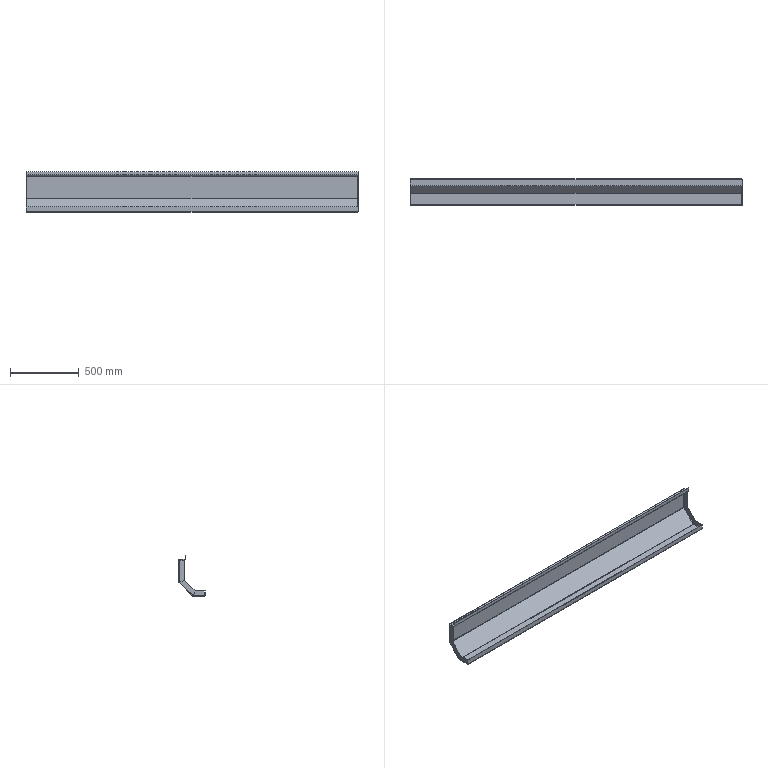Component | NX | UPPER_RIGHT_CROSSBEAM | 1 solid | 90 faces | volume 2507774 mm3 | plane 68 | cylinder 22 | commonest cylinder face diameters 10 x11 6 x11